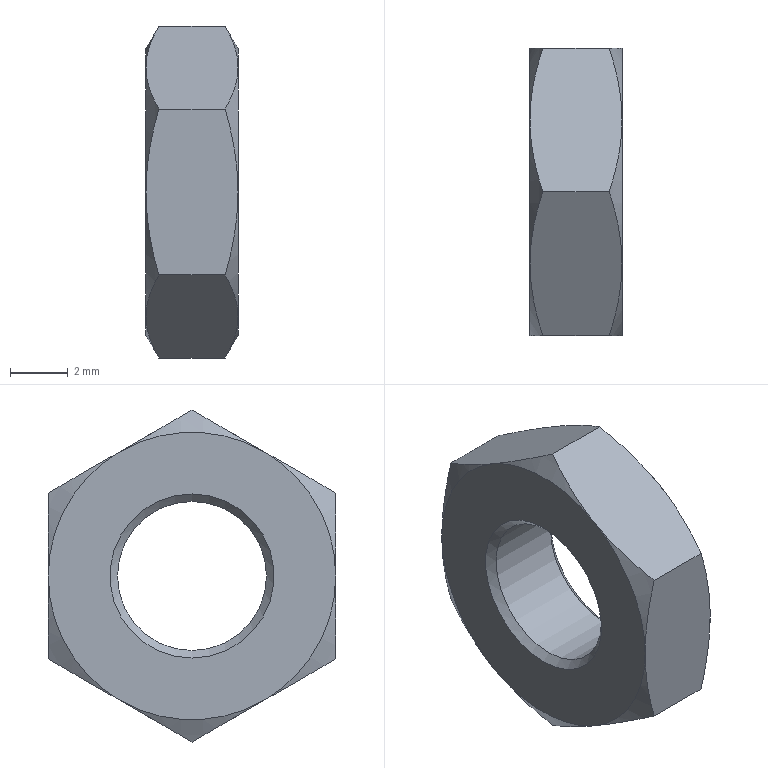Component | NX | GB-T6172_1-2000_M6X1 | 1 solid | 23 faces | volume 206 mm3 | cone 14 | plane 8 | cylinder 1 | commonest cylinder face diameters 5.188 x1